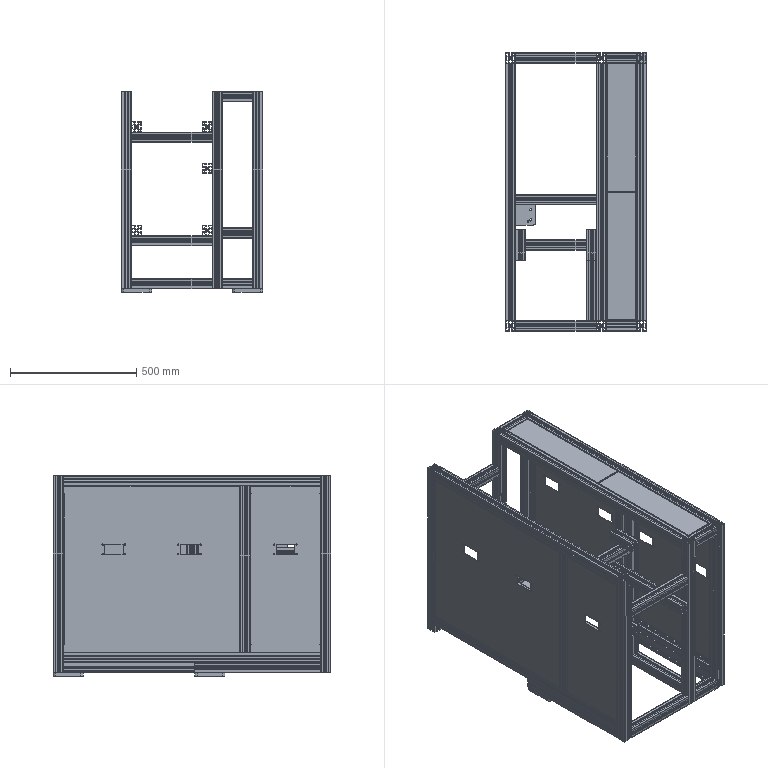Assembly | SolidWorks | mm | 41 component files | 41 solids | 3572 faces | box 560 x 1100 x 795 mm | volume 13071138 mm3 | plane 3042 | cylinder 514 | spline 16 | commonest cylinder face diameters 10.5 x170 6.8 x80 5 x56 8.5 x40 2 x36 0.762 x20 15 x20 9 x20
Bill of materials:
AluminumProfile120 | 9 | 6061 Alloy | Short straight prismatic bar with a constant square cross-section: four hollow square corner cells, a central round bore, diagonal webs, and a lengthwise slot open at the center of each of the four faces. The shortest of the profile bars in this set.
AluminumProfile320 | 6 | 6061 Alloy | Straight bar with the same four-slot square cross-section (hollow corner cells, central round bore, diagonal webs). Medium length.
AluminumProfile360 | 1 | 6061 Alloy | Straight bar with the shared four-slot square cross-section, shown with its long axis in a different orientation. Fairly long.
AluminumProfile480 | 1 | 6061 Alloy | Long straight bar with the shared four-slot square cross-section.
AluminumProfile500 | 1 | 6061 Alloy | Long straight bar with the shared four-slot square cross-section, shown in a different orientation from unnamed part.
AluminumProfile660 | 3 | 6061 Alloy | Long straight bar with the shared four-slot square cross-section, shown standing upright in the isometric view.
AluminumProfile720 | 5 | 6061 Alloy | The longest, most slender bar in the set, with the shared four-slot square cross-section.
AluminumProfile780 | 6 | 6061 Alloy | Long upright bar with the shared four-slot square cross-section, a little more slender than unnamed part.
AluminumProfileHFS8-4080Length720 | 1 | 1060 Alloy | Long straight prismatic bar with a constant rectangular cross-section, about 1:2 in aspect. The profile is a slotted extrusion-style section: two undercut T-shaped slots on each long side, one on each short side, two round center bores, an enclosed central cavity and four corner cavities.
CasterFixingPlate3 | 2 |  | Flat, thick square plate with rounded corners and nine plain round through-holes in two sizes, arranged in an asymmetric pattern.
SheetMetal120x510 | 2 |  | Long, shallow, thin-walled rectangular tray or cover: a flat, featureless top panel with short downturned flanges on all four edges. The flanges have open slots with rounded ends cut up from their free edges.
ThreeLowRackSidePlate1 | 2 | AISI 304 | Thin, flat rectangular panel, taller than it is wide (about 0.74:1). It has two rectangular through-cutouts side by side in the upper half, each with four small holes at its corners. Narrow edge returns or flanges run along two opposite edges.
ThreeLowRackSidePlate2 | 1 | AISI 304 | Thin, flat rectangular panel, a little wider than it is tall (about 1.06:1). Its features match unnamed part: two rectangular cutouts with four corner holes each, and narrow edge returns on two opposite edges.
ThreeLowRackSidePlate3 | 1 | AISI 304 | Thin, tall rectangular sheet-style panel with short bent-over flanges along its edges. It has one rectangular through-cutout centered side to side in the upper-middle area, with four small holes, one near each corner of the cutout.
Mates:
1. coincident | assembly face at (-24.557, -21.948, 2030) dir (-1, 0, 0) | assembly face at (-24.557, -1661.948, 1170) dir (-1, 0, 0)
2. coincident | assembly face at (-24.557, -21.948, 2030) dir (0, -1, 0) | assembly face at (15.443, -21.948, 1170) dir (0, 1, 0)
3. coincident | assembly face at (78.108, 18.052, 1170) dir (0, 0, 1) | assembly face at (-24.557, -1661.948, 1170) dir (0, 0, 1)
4. coincident | assembly face at (-24.557, -21.948, 2030) dir (-1, 0, 0) | assembly face at (-24.557, 898.052, 590) dir (-1, 0, 0)
5. coincident | assembly face at (-24.557, -21.948, 2030) dir (0, -1, 0) | assembly face at (15.443, -21.948, 692.665) dir (0, 1, 0)
6. distance | assembly face at (-24.557, 898.052, 630) dir (0, 0, 1) | assembly face at (-24.557, -1661.948, 1130) dir (0, 0, -1)
7. coincident | assembly face at (-24.557, -1661.948, 1170) dir (-1, 0, 0) | assembly face at (-24.557, -781.948, 2090) dir (-1, 0, 0)
8. coincident | assembly face at (-24.557, -1661.948, 1170) dir (0, 0, 1) | assembly face at (78.108, -741.948, 1170) dir (0, 0, 1)
9. coincident | assembly face at (15.443, -741.948, 1067.335) dir (0, -1, 0) | assembly face at (-24.557, -741.948, 2090) dir (0, 1, 0)
10. coincident | assembly face at (-24.557, -21.948, 2030) dir (0, -1, 0) | assembly face at (-1664.557, -21.948, 1130) dir (0, -1, 0)
11. coincident | assembly face at (-24.557, -21.948, 2030) dir (-1, 0, 0) | assembly face at (-24.557, 18.052, 1170) dir (1, 0, 0)
12. coincident | assembly face at (-24.557, -1661.948, 1170) dir (0, 0, 1) | assembly face at (-1664.557, 18.052, 1170) dir (0, 0, 1)
13. coincident | assembly face at (-24.557, -781.948, 2090) dir (0, -1, 0) | assembly face at (-1664.557, -781.948, 590) dir (0, -1, 0)
14. coincident | assembly face at (-24.557, -781.948, 2090) dir (-1, 0, 0) | assembly face at (-24.557, -741.948, 590) dir (1, 0, 0)
15. coincident | assembly face at (-24.557, 898.052, 630) dir (0, 0, 1) | assembly face at (-1664.557, -781.948, 630) dir (0, 0, 1)
16. coincident | assembly face at (-24.557, -781.948, 2090) dir (-1, 0, 0) | assembly face at (-24.557, 18.052, 527.335) dir (1, 0, 0)
17. coincident | assembly face at (-24.557, -21.948, 2030) dir (0, -1, 0) | assembly face at (1495.443, -21.948, 630) dir (0, -1, 0)
18. coincident | assembly face at (-24.557, 898.052, 630) dir (0, 0, 1) | assembly face at (1495.443, -21.948, 630) dir (0, 0, 1)
19. coincident | assembly face at (-24.557, -781.948, 2090) dir (0, -1, 0) | assembly face at (1495.443, -781.948, 1170) dir (0, -1, 0)
20. coincident | assembly face at (-24.557, -781.948, 2090) dir (-1, 0, 0) | assembly face at (-24.557, -741.948, 1067.335) dir (1, 0, 0)
21. coincident | assembly face at (-24.557, -1661.948, 1170) dir (0, 0, 1) | assembly face at (1495.443, -781.948, 1170) dir (0, 0, 1)
22. coincident | assembly face at (-1664.557, 18.052, 1170) dir (0, 0, 1) | assembly face at (-81.892, 18.052, 1170) dir (0, 0, 1)
23. coincident | assembly face at (-144.557, -84.613, 1170) dir (-1, 0, 0) | assembly face at (-144.557, -21.948, 2030) dir (1, 0, 0)
24. coincident | assembly face at (-1664.557, -21.948, 1130) dir (0, -1, 0) | assembly face at (-184.557, -21.948, 2030) dir (0, -1, 0)
25. coincident | assembly face at (-144.557, -741.948, 692.665) dir (-1, 0, 0) | assembly face at (-144.557, -781.948, 2030) dir (1, 0, 0)
26. coincident | assembly face at (-1664.557, -781.948, 590) dir (0, -1, 0) | assembly face at (-184.557, -781.948, 2030) dir (0, -1, 0)
27. coincident | assembly face at (1495.443, -781.948, 1170) dir (0, 0, 1) | assembly face at (-81.892, -741.948, 1170) dir (0, 0, 1)
28. coincident | assembly face at (-184.557, -741.948, 2030) dir (0, 1, 0) | assembly face at (-144.557, -741.948, 527.335) dir (0, -1, 0)
29. coincident | assembly face at (-184.557, -781.948, 2030) dir (-1, 0, 0) | assembly face at (-184.557, -1661.948, 630) dir (-1, 0, 0)
30. coincident | assembly face at (-1664.557, -781.948, 630) dir (0, 0, 1) | assembly face at (-184.557, -1661.948, 630) dir (0, 0, 1)
31. coincident | assembly face at (-184.557, -21.948, 2030) dir (-1, 0, 0) | assembly face at (-184.557, 898.052, 1170) dir (-1, 0, 0)
32. coincident | assembly face at (-184.557, -21.948, 2030) dir (0, -1, 0) | assembly face at (-81.892, -21.948, 1130) dir (0, 1, 0)
33. coincident | assembly face at (-1664.557, 18.052, 1170) dir (0, 0, 1) | assembly face at (-184.557, 898.052, 1170) dir (0, 0, 1)
34. coincident | assembly face at (-184.557, -781.948, 2030) dir (-1, 0, 0) | assembly face at (-184.557, -741.948, 590) dir (1, 0, 0)
35. coincident | assembly face at (-184.557, -781.948, 2030) dir (0, -1, 0) | assembly face at (-1824.557, -781.948, 590) dir (0, -1, 0)
36. coincident | assembly face at (-184.557, -1661.948, 630) dir (0, 0, 1) | assembly face at (-1824.557, -781.948, 630) dir (0, 0, 1)
37. coincident | assembly face at (-184.557, -21.948, 2030) dir (-1, 0, 0) | assembly face at (-184.557, 18.052, 630) dir (1, 0, 0)
38. coincident | assembly face at (-184.557, -21.948, 2030) dir (0, -1, 0) | assembly face at (-1824.557, -21.948, 590) dir (0, -1, 0)
39. coincident | assembly face at (-184.557, -1661.948, 630) dir (0, 0, 1) | assembly face at (-1824.557, 18.052, 630) dir (0, 0, 1)
40. coincident | assembly face at (-184.557, -21.948, 2030) dir (-1, 0, 0) | assembly face at (-184.557, 18.052, 970) dir (1, 0, 0)
41. coincident | assembly face at (-184.557, -21.948, 2030) dir (0, -1, 0) | assembly face at (-1824.557, -21.948, 970) dir (0, -1, 0)
42. distance | assembly face at (-1664.557, 18.052, 1170) dir (0, 0, 1) | assembly face at (-1824.557, -21.948, 1010) dir (0, 0, 1)
43. coincident | assembly face at (-184.557, -781.948, 2030) dir (0, -1, 0) | assembly face at (-1824.557, -781.948, 970) dir (0, -1, 0)
44. coincident | assembly face at (-184.557, -781.948, 2030) dir (-1, 0, 0) | assembly face at (-184.557, -741.948, 1010) dir (1, 0, 0)
45. distance | assembly face at (-184.557, 898.052, 1170) dir (0, 0, 1) | assembly face at (-1824.557, -741.948, 1010) dir (0, 0, 1)
46. coincident | assembly face at (-184.557, -21.948, 2030) dir (-1, 0, 0) | assembly face at (-184.557, 1578.052, 1050) dir (1, 0, 0)
47. coincident | assembly face at (-1824.557, -21.948, 1010) dir (0, 0, 1) | assembly face at (-224.557, 1578.052, 1010) dir (0, 0, -1)
48. distance | assembly face at (-224.557, -61.948, 1010) dir (0, -1, 0) | assembly face at (-1824.557, -21.948, 970) dir (0, -1, 0)
49. coincident | assembly face at (-464.557, 18.052, 1072.665) dir (-1, 0, 0) | assembly face at (-464.557, -1581.948, 1010) dir (-1, 0, 0)
50. coincident | assembly face at (-1824.557, -21.948, 1010) dir (0, 0, 1) | assembly face at (-464.557, -1581.948, 1010) dir (0, 0, -1)
51. distance | assembly face at (-464.557, 58.052, 1050) dir (0, 1, 0) | assembly face at (-1824.557, 18.052, 970) dir (0, 1, 0)
52. coincident | assembly face at (-184.557, -781.948, 2030) dir (-1, 0, 0) | assembly face at (-184.557, -2341.948, 1010) dir (1, 0, 0)
53. coincident | assembly face at (-1824.557, -741.948, 1010) dir (0, 0, 1) | assembly face at (-224.557, -2341.948, 1010) dir (0, 0, -1)
54. distance | assembly face at (-224.557, -701.948, 1050) dir (0, 1, 0) | assembly face at (-1824.557, -741.948, 970) dir (0, 1, 0)
55. coincident | assembly face at (-464.557, -844.613, 1010) dir (-1, 0, 0) | assembly face at (-464.557, 818.052, 1010) dir (-1, 0, 0)
56. coincident | assembly face at (-1824.557, -741.948, 1010) dir (0, 0, 1) | assembly face at (-464.557, 818.052, 1010) dir (0, 0, -1)
57. distance | assembly face at (-424.557, -821.948, 1010) dir (0, -1, 0) | assembly face at (-1824.557, -781.948, 970) dir (0, -1, 0)
58. coincident | assembly face at (-184.557, -21.948, 2030) dir (-1, 0, 0) | assembly face at (-184.557, -1581.948, 630) dir (1, 0, 0)
59. coincident | assembly face at (-1824.557, 18.052, 630) dir (0, 0, 1) | assembly face at (-184.557, -1581.948, 630) dir (0, 0, -1)
60. distance | assembly face at (-1824.557, 18.052, 590) dir (0, 1, 0) | assembly face at (-224.557, 58.052, 630) dir (0, 1, 0)
61. coincident | assembly face at (-464.557, -84.613, 630) dir (-1, 0, 0) | assembly face at (-464.557, -1581.948, 630) dir (-1, 0, 0)
62. coincident | assembly face at (-1824.557, 18.052, 630) dir (0, 0, 1) | assembly face at (-464.557, -1581.948, 630) dir (0, 0, -1)
63. distance | assembly face at (-464.557, 58.052, 670) dir (0, 1, 0) | assembly face at (-1824.557, 18.052, 590) dir (0, 1, 0)
64. coincident | assembly face at (-184.557, -781.948, 2030) dir (-1, 0, 0) | assembly face at (-184.557, 818.052, 630) dir (1, 0, 0)
65. coincident | assembly face at (-1824.557, -781.948, 630) dir (0, 0, 1) | assembly face at (-224.557, 818.052, 630) dir (0, 0, -1)
66. distance | assembly face at (-1824.557, -781.948, 590) dir (0, -1, 0) | assembly face at (-184.557, -821.948, 630) dir (0, -1, 0)
67. coincident | assembly face at (-464.557, -741.948, 692.665) dir (-1, 0, 0) | assembly face at (-464.557, -2341.948, 630) dir (-1, 0, 0)
68. coincident | assembly face at (-1824.557, -781.948, 630) dir (0, 0, 1) | assembly face at (-464.557, -2341.948, 630) dir (0, 0, -1)
69. distance | assembly face at (-1824.557, -741.948, 590) dir (0, 1, 0) | assembly face at (-464.557, -701.948, 670) dir (0, 1, 0)
70. coincident | assembly face at (-464.557, -1581.948, 1010) dir (-1, 0, 0) | assembly face at (-464.557, -21.948, 2390) dir (-1, 0, 0)
71. coincident | assembly face at (-1824.557, -21.948, 970) dir (0, -1, 0) | assembly face at (-464.557, -21.948, 2390) dir (0, -1, 0)
72. coincident | assembly face at (-1824.557, -21.948, 970) dir (0, 0, -1) | assembly face at (-361.892, 18.052, 970) dir (0, 0, 1)
73. coincident | assembly face at (-464.557, -844.613, 1010) dir (-1, 0, 0) | assembly face at (-464.557, -781.948, 2390) dir (-1, 0, 0)
74. coincident | assembly face at (-1824.557, -781.948, 970) dir (0, -1, 0) | assembly face at (-464.557, -781.948, 2390) dir (0, -1, 0)
75. coincident | assembly face at (-1824.557, -741.948, 970) dir (0, 0, -1) | assembly face at (-361.892, -741.948, 970) dir (0, 0, 1)
76. coincident | assembly face at (-464.557, -741.948, 692.665) dir (-1, 0, 0) | assembly face at (-464.557, -781.948, 2030) dir (-1, 0, 0)
77. coincident | assembly face at (-1824.557, -781.948, 590) dir (0, -1, 0) | assembly face at (-464.557, -781.948, 2030) dir (0, -1, 0)
78. coincident | assembly face at (-1824.557, -781.948, 590) dir (0, 0, -1) | assembly face at (-361.892, -741.948, 590) dir (0, 0, 1)
79. coincident | assembly face at (-464.557, -84.613, 630) dir (-1, 0, 0) | assembly face at (-464.557, -21.948, 2030) dir (-1, 0, 0)
80. coincident | assembly face at (-1824.557, 18.052, 590) dir (0, 1, 0) | assembly face at (-464.557, 18.052, 2030) dir (0, 1, 0)
81. coincident | assembly face at (-1824.557, 18.052, 590) dir (0, 0, -1) | assembly face at (-361.892, 18.052, 590) dir (0, 0, 1)
82. coincident | assembly face at (-24.557, -741.948, 1067.335) dir (1, 0, 0) | assembly face at (-24.557, -781.948, 2030) dir (-1, 0, 0)
83. coincident | assembly face at (1495.443, -781.948, 1170) dir (0, -1, 0) | assembly face at (-24.557, -781.948, 2030) dir (0, -1, 0)
84. coincident | assembly face at (1495.443, -781.948, 1170) dir (0, 0, 1) | assembly face at (78.108, -741.948, 1170) dir (0, 0, 1)
85. coincident | assembly face at (15.443, -781.948, 2030) dir (1, 0, 0) | assembly face at (15.443, -631.948, 375) dir (1, 0, 0)
86. coincident | assembly face at (-24.557, -781.948, 2030) dir (0, -1, 0) | assembly face at (15.443, -781.948, 375) dir (0, -1, 0)
87. coincident | assembly face at (-24.557, -741.948, 390) dir (0, 0, -1) | assembly face at (15.443, -631.948, 390) dir (0, 0, 1)
88. coincident | assembly face at (15.443, -21.948, 2030) dir (1, 0, 0) | assembly face at (15.443, 18.052, 375) dir (1, 0, 0)
89. coincident | assembly face at (-24.557, 18.052, 2030) dir (0, 1, 0) | assembly face at (15.443, 18.052, 375) dir (0, 1, 0)
90. coincident | assembly face at (-24.557, 18.052, 390) dir (0, 0, -1) | assembly face at (15.443, 18.052, 390) dir (0, 0, 1)
91. coincident | assembly face at (-464.557, -21.948, 2030) dir (-1, 0, 0) | assembly face at (-464.557, -131.948, 375) dir (-1, 0, 0)
92. coincident | assembly face at (-464.557, 18.052, 2030) dir (0, 1, 0) | assembly face at (-464.557, 18.052, 375) dir (0, 1, 0)
93. coincident | assembly face at (-464.557, 18.052, 390) dir (0, 0, -1) | assembly face at (-464.557, -131.948, 390) dir (0, 0, 1)
94. coincident | assembly face at (-464.557, -781.948, 2030) dir (0, -1, 0) | assembly face at (-464.557, -781.948, 375) dir (0, -1, 0)
95. coincident | assembly face at (-464.557, -781.948, 2030) dir (-1, 0, 0) | assembly face at (-464.557, -781.948, 375) dir (-1, 0, 0)
96. coincident | assembly face at (-464.557, -741.948, 390) dir (0, 0, -1) | assembly face at (-464.557, -781.948, 390) dir (0, 0, 1)
97. coincident | assembly face at (-24.557, -741.948, 590) dir (1, 0, 0) | assembly face at (-24.557, -781.948, 2030) dir (-1, 0, 0)
98. coincident | assembly face at (-184.557, -781.948, 2030) dir (-1, 0, 0) | assembly face at (-184.557, 898.052, 1170) dir (-1, 0, 0)
99. coincident | assembly face at (1495.443, -781.948, 1170) dir (0, -1, 0) | assembly face at (-184.557, -781.948, 2030) dir (0, -1, 0)
100. coincident | assembly face at (15.443, -741.948, 1067.335) dir (0, -1, 0) | assembly face at (-24.557, -741.948, 2030) dir (0, 1, 0)
101. coincident | assembly face at (-184.557, -1661.948, 630) dir (-1, 0, 0) | assembly face at (-184.557, 898.052, 1170) dir (-1, 0, 0)
102. coincident | assembly face at (1495.443, -21.948, 630) dir (0, 0, 1) | assembly face at (-184.557, -1661.948, 630) dir (0, 0, 1)
103. distance | assembly face at (-184.557, -1661.948, 590) dir (0, 0, -1) | assembly face at (-24.557, -741.948, 390) dir (0, 0, -1)
104. coincident | assembly face at (-24.557, -741.948, 2030) dir (0, 1, 0) | assembly face at (-4.557, -741.948, 430) dir (0, -1, 0)
105. coincident | assembly face at (15.443, -781.948, 2030) dir (1, 0, 0) | assembly face at (15.443, -741.948, 415.3) dir (1, 0, 0)
106. coincident | assembly face at (-24.557, -741.948, 390) dir (0, 0, -1) | assembly face at (0.7428, -741.948, 390) dir (0, 0, -1)
107. coincident | AluminumProfile780-1 face at (-768.352, 51.783, 1543.715) dir (-1, 0, 0) | AluminumProfile720-1 face at (-768.352, 671.783, 643.715) dir (-1, 0, 0)
108. coincident | AluminumProfile780-1 face at (-768.352, 51.783, 1543.715) dir (0, -1, 0) | AluminumProfile720-1 face at (-831.017, 51.783, 683.715) dir (0, 1, 0)
109. coincident | AluminumProfile780-1 face at (-665.687, 91.783, 683.715) dir (0, 0, 1) | AluminumProfile720-1 face at (-728.352, 671.783, 683.715) dir (0, 0, 1)
110. coincident | AluminumProfile780-1 face at (-768.352, 51.783, 1543.715) dir (0, -1, 0) | assembly face at (-748.352, 51.783, -56.285) dir (0, 1, 0)
111. coincident | AluminumProfile780-1 face at (-768.352, 51.783, 1543.715) dir (-1, 0, 0) | assembly face at (-768.352, 51.783, -70.985) dir (-1, 0, 0)
112. coincident | AluminumProfile780-1 face at (-768.352, 91.783, -96.285) dir (0, 0, -1) | assembly face at (-753.652, 51.783, -96.285) dir (0, 0, -1)
113. coincident | AluminumProfile720-1 face at (-728.352, -968.217, 683.715) dir (0, -1, 0) | AluminumProfile780-2 face at (-768.352, -968.217, 1543.715) dir (0, 1, 0)
114. coincident | AluminumProfile720-1 face at (-768.352, 671.783, 643.715) dir (-1, 0, 0) | AluminumProfile780-2 face at (-768.352, -1008.217, 1543.715) dir (-1, 0, 0)
115. coincident | AluminumProfile720-1 face at (-728.352, 671.783, 683.715) dir (0, 0, 1) | AluminumProfile780-2 face at (-665.687, -968.217, 683.715) dir (0, 0, 1)
116. coincident | AluminumProfile780-1 face at (-768.352, 51.783, 1543.715) dir (0, -1, 0) | AluminumProfileHFS8-4080Length720-2 face at (-748.352, 51.783, -56.285) dir (0, 1, 0)
117. coincident | AluminumProfile780-1 face at (-768.352, 51.783, 1543.715) dir (-1, 0, 0) | AluminumProfileHFS8-4080Length720-2 face at (-768.352, 51.783, -70.985) dir (-1, 0, 0)
118. coincident | AluminumProfile780-1 face at (-768.352, 91.783, -96.285) dir (0, 0, -1) | AluminumProfileHFS8-4080Length720-2 face at (-753.652, 51.783, -96.285) dir (0, 0, -1)
119. coincident | AluminumProfile780-1 face at (-768.352, 51.783, 1543.715) dir (-1, 0, 0) | AluminumProfile120-1 face at (-768.352, 91.783, 643.715) dir (1, 0, 0)
120. coincident | AluminumProfile720-1 face at (-728.352, 671.783, 683.715) dir (0, 0, 1) | AluminumProfile120-1 face at (-2408.352, 51.783, 683.715) dir (0, 0, 1)
121. coincident | AluminumProfile780-1 face at (-768.352, 91.783, 1543.715) dir (0, 1, 0) | AluminumProfile120-1 face at (-2408.352, 91.783, 643.715) dir (0, 1, 0)
122. coincident | AluminumProfileHFS8-4080Length720-2 face at (-768.352, 51.783, -70.985) dir (-1, 0, 0) | AluminumProfile120-2 face at (-768.352, -1008.217, 643.715) dir (1, 0, 0)
123. coincident | AluminumProfile720-1 face at (-728.352, 671.783, 683.715) dir (0, 0, 1) | AluminumProfile120-2 face at (-2408.352, -1008.217, 683.715) dir (0, 0, 1)
124. coincident | AluminumProfile780-2 face at (-768.352, -1008.217, 1543.715) dir (0, -1, 0) | AluminumProfile120-2 face at (-2408.352, -1008.217, 683.715) dir (0, -1, 0)
125. coincident | AluminumProfile780-1 face at (-768.352, 51.783, 1543.715) dir (-1, 0, 0) | AluminumProfile120-3 face at (-768.352, 91.783, 143.715) dir (1, 0, 0)
126. coincident | AluminumProfile780-1 face at (-768.352, 51.783, 1543.715) dir (0, -1, 0) | AluminumProfile120-3 face at (-2408.352, 51.783, 103.715) dir (0, -1, 0)
127. distance | AluminumProfileHFS8-4080Length720-2 face at (-753.652, 51.783, -96.285) dir (0, 0, -1) | AluminumProfile120-3 face at (-2408.352, 91.783, 103.715) dir (0, 0, -1)
128. coincident | AluminumProfile780-2 face at (-768.352, -1008.217, 1543.715) dir (-1, 0, 0) | AluminumProfile120-4 face at (-768.352, -968.217, -158.95) dir (1, 0, 0)
129. coincident | AluminumProfile780-2 face at (-768.352, -1008.217, 1543.715) dir (0, -1, 0) | AluminumProfile120-4 face at (751.648, -1008.217, -56.285) dir (0, -1, 0)
130. coincident | AluminumProfileHFS8-4080Length720-2 face at (-753.652, 51.783, -96.285) dir (0, 0, -1) | AluminumProfile120-4 face at (751.648, -1008.217, -96.285) dir (0, 0, -1)
131. coincident | AluminumProfile120-4 face at (751.648, -1008.217, -56.285) dir (0, -1, 0) | AluminumProfile780-3 face at (-928.352, -1008.217, 1543.715) dir (0, -1, 0)
132. coincident | AluminumProfile120-4 face at (-888.352, -968.217, -56.285) dir (-1, 0, 0) | AluminumProfile780-3 face at (-888.352, -1008.217, 1543.715) dir (1, 0, 0)
133. coincident | AluminumProfile120-2 face at (-2408.352, -1008.217, 683.715) dir (0, 0, 1) | AluminumProfile780-3 face at (-825.687, -968.217, 683.715) dir (0, 0, 1)
134. coincident | AluminumProfile120-3 face at (-888.352, -10.882, 143.715) dir (-1, 0, 0) | AluminumProfile780-4 face at (-888.352, 51.783, 1543.715) dir (1, 0, 0)
135. coincident | AluminumProfile120-3 face at (-2408.352, 91.783, 103.715) dir (0, 1, 0) | AluminumProfile780-4 face at (-928.352, 91.783, 1543.715) dir (0, 1, 0)
136. coincident | AluminumProfile120-1 face at (-2408.352, 51.783, 683.715) dir (0, 0, 1) | AluminumProfile780-4 face at (-825.687, 91.783, 683.715) dir (0, 0, 1)
137. coincident | AluminumProfile780-3 face at (-928.352, -968.217, 1543.715) dir (0, 1, 0) | AluminumProfile720-2 face at (-825.687, -968.217, 683.715) dir (0, -1, 0)
138. coincident | AluminumProfile780-3 face at (-928.352, -1008.217, 1543.715) dir (-1, 0, 0) | AluminumProfile720-2 face at (-928.352, -1588.217, 643.715) dir (-1, 0, 0)
139. coincident | AluminumProfile120-2 face at (-2408.352, -1008.217, 683.715) dir (0, 0, 1) | AluminumProfile720-2 face at (-928.352, -1588.217, 683.715) dir (0, 0, 1)
140. coincident | AluminumProfile780-4 face at (-928.352, 51.783, 1543.715) dir (0, -1, 0) | assembly face at (-928.352, 51.783, 143.715) dir (0, 1, 0)
141. coincident | AluminumProfile780-3 face at (-928.352, -1008.217, 1543.715) dir (-1, 0, 0) | assembly face at (-928.352, -1588.217, 103.715) dir (-1, 0, 0)
142. coincident | AluminumProfile120-4 face at (751.648, -1008.217, -96.285) dir (0, 0, -1) | assembly face at (-928.352, -1588.217, 103.715) dir (0, 0, -1)
143. coincident | AluminumProfile780-3 face at (-928.352, -1008.217, 1543.715) dir (0, -1, 0) | assembly face at (311.648, -708.217, 143.715) dir (0, -1, 0)
144. coincident | AluminumProfile780-3 face at (-928.352, -1008.217, 1543.715) dir (-1, 0, 0) | assembly face at (-928.352, -668.217, 41.05) dir (1, 0, 0)
145. coincident | AluminumProfile120-4 face at (751.648, -1008.217, -56.285) dir (0, 0, 1) | assembly face at (311.648, -708.217, 143.715) dir (0, 0, 1)
146. coincident | AluminumProfile780-3 face at (-928.352, -1008.217, 1543.715) dir (-1, 0, 0) | assembly face at (-928.352, 946.601, 143.715) dir (1, 0, 0)
147. distance | assembly face at (-928.352, -748.217, 143.715) dir (0, -1, 0) | assembly face at (311.648, -708.217, 143.715) dir (0, -1, 0)
148. coincident | assembly face at (311.648, -708.217, 143.715) dir (0, 0, 1) | assembly face at (-968.352, 891.783, 143.715) dir (0, 0, -1)
149. coincident | assembly face at (-928.352, -693.399, 143.715) dir (0, -1, 0) | assembly face at (-1105.687, -693.399, 183.715) dir (0, -1, 0)
150. coincident | assembly face at (-968.352, 946.601, 183.715) dir (0, 0, 1) | assembly face at (-1208.352, -2213.399, 183.715) dir (0, 0, 1)
151. distance | assembly face at (-968.352, 946.601, 143.715) dir (-1, 0, 0) | assembly face at (-1168.352, -2213.399, 143.715) dir (1, 0, 0)
152. coincident | AluminumProfile780-3 face at (-928.352, -1008.217, 1543.715) dir (-1, 0, 0) | assembly face at (-928.352, -668.217, 523.715) dir (1, 0, 0)
153. coincident | AluminumProfile780-3 face at (-928.352, -1008.217, 1543.715) dir (0, -1, 0) | assembly face at (-2568.352, -708.217, 483.715) dir (0, -1, 0)
154. distance | AluminumProfile720-2 face at (-928.352, -1588.217, 683.715) dir (0, 0, 1) | assembly face at (-2568.352, -668.217, 523.715) dir (0, 0, 1)
155. coincident | assembly face at (-928.352, -748.217, 143.715) dir (0, -1, 0) | assembly face at (-865.687, -748.217, 563.715) dir (0, -1, 0)
156. coincident | AluminumProfile780-3 face at (-928.352, -1008.217, 1543.715) dir (-1, 0, 0) | assembly face at (-928.352, -2268.217, 523.715) dir (1, 0, 0)
157. coincident | assembly face at (-2568.352, -668.217, 523.715) dir (0, 0, 1) | assembly face at (-968.352, -2268.217, 523.715) dir (0, 0, -1)
158. coincident | assembly face at (-865.687, -748.217, 563.715) dir (0, -1, 0) | assembly face at (-1208.352, -748.217, 626.38) dir (0, -1, 0)
159. coincident | assembly face at (-968.352, -2268.217, 563.715) dir (0, 0, 1) | assembly face at (-1168.352, -2268.217, 563.715) dir (0, 0, 1)
160. distance | assembly face at (-968.352, -2268.217, 523.715) dir (-1, 0, 0) | assembly face at (-1168.352, -2268.217, 523.715) dir (1, 0, 0)
161. coincident | AluminumProfile780-3 face at (-928.352, -1008.217, 1543.715) dir (0, -1, 0) | AluminumProfile320-1 face at (-2568.352, -1008.217, -96.285) dir (0, -1, 0)
162. coincident | AluminumProfile780-3 face at (-928.352, -1008.217, 1543.715) dir (-1, 0, 0) | AluminumProfile320-1 face at (-928.352, -968.217, -56.285) dir (1, 0, 0)
163. coincident | AluminumProfile780-3 face at (-928.352, -1008.217, 1543.715) dir (0, -1, 0) | AluminumProfile320-2 face at (-2568.352, -1008.217, 483.715) dir (0, -1, 0)
164. coincident | AluminumProfile780-3 face at (-928.352, -1008.217, 1543.715) dir (-1, 0, 0) | AluminumProfile320-2 face at (-928.352, -968.217, 523.715) dir (1, 0, 0)
165. distance | AluminumProfile720-2 face at (-928.352, -1588.217, 683.715) dir (0, 0, 1) | AluminumProfile320-2 face at (-2568.352, -968.217, 523.715) dir (0, 0, 1)
166. coincident | AluminumProfile780-4 face at (-928.352, 91.783, 1543.715) dir (0, 1, 0) | AluminumProfile320-3 face at (-2568.352, 91.783, -96.285) dir (0, 1, 0)
167. coincident | AluminumProfile780-4 face at (-928.352, 51.783, 1543.715) dir (-1, 0, 0) | AluminumProfile320-3 face at (-928.352, 91.783, -96.285) dir (1, 0, 0)
168. coincident | AluminumProfile780-4 face at (-928.352, 51.783, 1543.715) dir (-1, 0, 0) | AluminumProfile320-4 face at (-928.352, 91.783, 483.715) dir (1, 0, 0)
169. coincident | AluminumProfile780-4 face at (-928.352, 91.783, 1543.715) dir (0, 1, 0) | AluminumProfile320-4 face at (-2568.352, 91.783, 483.715) dir (0, 1, 0)
170. distance | AluminumProfile720-2 face at (-928.352, -1588.217, 683.715) dir (0, 0, 1) | AluminumProfile320-4 face at (-2568.352, 51.783, 523.715) dir (0, 0, 1)
171. coincident | AluminumProfile780-4 face at (-928.352, 51.783, 1543.715) dir (-1, 0, 0) | assembly face at (-928.352, -1508.217, 523.715) dir (1, 0, 0)
172. coincident | AluminumProfile320-4 face at (-2568.352, 51.783, 523.715) dir (0, 0, 1) | assembly face at (-928.352, -1508.217, 523.715) dir (0, 0, -1)
173. distance | assembly face at (-968.352, 131.783, 523.715) dir (0, 1, 0) | AluminumProfile320-4 face at (-2568.352, 91.783, 483.715) dir (0, 1, 0)
174. coincident | AluminumProfile780-3 face at (-928.352, -1008.217, 1543.715) dir (-1, 0, 0) | assembly face at (-928.352, -2268.217, 523.715) dir (1, 0, 0)
175. distance | assembly face at (-968.352, -628.217, 523.715) dir (0, 1, 0) | AluminumProfile320-2 face at (-2568.352, -968.217, 483.715) dir (0, 1, 0)
176. coincident | AluminumProfile320-2 face at (-2568.352, -968.217, 523.715) dir (0, 0, 1) | assembly face at (-928.352, -2268.217, 523.715) dir (0, 0, -1)
177. coincident | assembly face at (-968.352, -748.217, 626.38) dir (0, -1, 0) | assembly face at (-1208.352, -748.217, 626.38) dir (0, -1, 0)
178. coincident | AluminumProfile320-2 face at (-2568.352, -968.217, 523.715) dir (0, 0, 1) | assembly face at (-1168.352, -2268.217, 523.715) dir (0, 0, -1)
179. distance | assembly face at (-968.352, -2268.217, 523.715) dir (-1, 0, 0) | assembly face at (-1168.352, -2268.217, 523.715) dir (1, 0, 0)
180. coincident | AluminumProfile780-3 face at (-928.352, -1008.217, 1543.715) dir (-1, 0, 0) | assembly face at (-928.352, -2268.217, 143.715) dir (1, 0, 0)
181. coincident | AluminumProfile320-1 face at (-2568.352, -968.217, -56.285) dir (0, 0, 1) | assembly face at (-968.352, -2268.217, 143.715) dir (0, 0, -1)
182. distance | AluminumProfile320-1 face at (-2568.352, -968.217, -96.285) dir (0, 1, 0) | assembly face at (-968.352, -628.217, 183.715) dir (0, 1, 0)
183. coincident | AluminumProfile780-4 face at (-928.352, 51.783, 1543.715) dir (-1, 0, 0) | assembly face at (-928.352, -1508.217, 143.715) dir (1, 0, 0)
184. distance | assembly face at (-968.352, 131.783, 183.715) dir (0, 1, 0) | AluminumProfile320-3 face at (-2568.352, 91.783, -96.285) dir (0, 1, 0)
185. coincident | AluminumProfile320-3 face at (-2568.352, 51.783, -56.285) dir (0, 0, 1) | assembly face at (-1208.352, 1651.783, 143.715) dir (0, 0, -1)
186. distance | assembly face at (-968.352, -1508.217, 143.715) dir (-1, 0, 0) | assembly face at (-1168.352, 1651.783, 143.715) dir (1, 0, 0)
187. distance | assembly face at (-1168.352, 11.783, 143.715) dir (0, -1, 0) | AluminumProfile320-3 face at (-2568.352, 51.783, -96.285) dir (0, -1, 0)
188. coincident | AluminumProfile320-4 face at (-2568.352, 51.783, 523.715) dir (0, 0, 1) | assembly face at (-1208.352, -1508.217, 523.715) dir (0, 0, -1)
189. distance | assembly face at (-1208.352, 131.783, 563.715) dir (0, 1, 0) | AluminumProfile320-4 face at (-2568.352, 91.783, 483.715) dir (0, 1, 0)
190. distance | assembly face at (-968.352, -1508.217, 523.715) dir (-1, 0, 0) | assembly face at (-1168.352, -1508.217, 523.715) dir (1, 0, 0)
191. coincident | AluminumProfile320-1 face at (-2568.352, -968.217, -56.285) dir (0, 0, 1) | assembly face at (-1208.352, -2268.217, 143.715) dir (0, 0, -1)
192. distance | AluminumProfile320-1 face at (-2568.352, -968.217, -96.285) dir (0, 1, 0) | assembly face at (-1208.352, -628.217, 183.715) dir (0, 1, 0)
193. distance | assembly face at (-968.352, -2268.217, 143.715) dir (-1, 0, 0) | assembly face at (-1168.352, -2268.217, 143.715) dir (1, 0, 0)
194. coincident | AluminumProfile320-1 face at (-2568.352, -1008.217, -96.285) dir (0, -1, 0) | AluminumProfile780-5 face at (-1288.352, -1008.217, 1543.715) dir (0, -1, 0)
195. coincident | AluminumProfile320-1 face at (-1248.352, -1070.882, -56.285) dir (-1, 0, 0) | AluminumProfile780-5 face at (-1248.352, -1008.217, 1543.715) dir (1, 0, 0)
196. coincident | AluminumProfile780-3 face at (-928.352, -968.217, -96.285) dir (0, 0, -1) | AluminumProfile780-5 face at (-1288.352, -968.217, -96.285) dir (0, 0, -1)
197. coincident | AluminumProfile320-3 face at (-1248.352, 91.783, 6.38) dir (-1, 0, 0) | AluminumProfile780-6 face at (-1248.352, 51.783, 1543.715) dir (1, 0, 0)
198. coincident | AluminumProfile320-3 face at (-2568.352, 91.783, -96.285) dir (0, 1, 0) | AluminumProfile780-6 face at (-1288.352, 91.783, 1543.715) dir (0, 1, 0)
199. coincident | AluminumProfile780-4 face at (-928.352, 91.783, -96.285) dir (0, 0, -1) | AluminumProfile780-6 face at (-1288.352, 91.783, -96.285) dir (0, 0, -1)
200. coincident | AluminumProfile780-6 face at (-1288.352, 51.783, 1543.715) dir (0, -1, 0) | AluminumProfile720-4 face at (-1248.352, 51.783, 746.38) dir (0, 1, 0)
201. coincident | AluminumProfile780-6 face at (-1288.352, 51.783, 1543.715) dir (-1, 0, 0) | AluminumProfile720-4 face at (-1288.352, 671.783, 643.715) dir (-1, 0, 0)
202. coincident | AluminumProfile780-6 face at (-1185.687, 91.783, 683.715) dir (0, 0, 1) | AluminumProfile720-4 face at (-1288.352, 671.783, 683.715) dir (0, 0, 1)
203. coincident | AluminumProfile780-6 face at (-1288.352, 51.783, 1543.715) dir (-1, 0, 0) | assembly face at (-1288.352, 971.783, 103.715) dir (-1, 0, 0)
204. coincident | AluminumProfile780-6 face at (-1288.352, 51.783, 1543.715) dir (0, -1, 0) | assembly face at (-1248.352, 51.783, 206.38) dir (0, 1, 0)
205. coincident | AluminumProfile320-3 face at (-2568.352, 51.783, -56.285) dir (0, 0, 1) | assembly face at (-1288.352, 971.783, 143.715) dir (0, 0, 1)
206. coincident | AluminumProfile720-4 face at (-1288.352, 671.783, 643.715) dir (0, 0, -1) | assembly face at (-1185.687, -468.217, 643.715) dir (0, 0, 1)
207. coincident | AluminumProfile720-4 face at (-1288.352, 671.783, 643.715) dir (-1, 0, 0) | assembly face at (-1288.352, -508.217, 1783.715) dir (-1, 0, 0)
208. distance | AluminumProfile720-2 face at (-928.352, -1588.217, 683.715) dir (0, 0, 1) | assembly face at (-2568.352, -768.217, 523.715) dir (0, 0, 1)
209. coincident | assembly face at (-2568.352, -768.217, 523.715) dir (0, 0, 1) | assembly face at (-968.352, 791.783, 523.715) dir (0, 0, -1)
210. distance | assembly face at (-2568.352, -808.217, 483.715) dir (0, -1, 0) | assembly face at (-928.352, -848.217, 523.715) dir (0, -1, 0)
211. coincident | assembly face at (-928.352, -1588.217, 103.715) dir (-1, 0, 0) | assembly face at (-928.352, -2368.217, 143.715) dir (1, 0, 0)
212. coincident | assembly face at (-2568.352, -768.217, 143.715) dir (0, 0, 1) | assembly face at (-928.352, -2368.217, 143.715) dir (0, 0, -1)
213. distance | assembly face at (-968.352, -728.217, 143.715) dir (0, 1, 0) | assembly face at (-2568.352, -768.217, 103.715) dir (0, 1, 0)
214. distance | assembly face at (-968.352, -2368.217, 143.715) dir (-1, 0, 0) | assembly face at (-1168.352, -2368.217, 143.715) dir (1, 0, 0)
215. coincident | assembly face at (-968.352, 791.783, 563.715) dir (0, 0, 1) | assembly face at (-1208.352, -2368.217, 563.715) dir (0, 0, 1)
216. coincident | assembly face at (-928.352, -848.217, 523.715) dir (0, -1, 0) | assembly face at (-1105.687, -848.217, 563.715) dir (0, -1, 0)
217. coincident | assembly face at (-1168.352, -2147.847, 143.715) dir (1, 0, 0) | assembly face at (-1168.352, -2368.217, 523.715) dir (1, 0, 0)
218. coincident | assembly face at (-928.352, -1588.217, 103.715) dir (0, 0, -1) | assembly face at (-2568.352, -653.542, 103.715) dir (0, 0, -1)
219. coincident | AluminumProfile720-6 face at (-1248.352, -968.217, -56.285) dir (0, -1, 0) | AluminumProfile780-5 face at (-1288.352, -968.217, 1543.715) dir (0, 1, 0)
220. coincident | AluminumProfile780-5 face at (-1288.352, -1008.217, 1543.715) dir (-1, 0, 0) | AluminumProfile720-6 face at (-1288.352, 671.783, -56.285) dir (-1, 0, 0)
221. distance | AluminumProfile780-6 face at (-1288.352, 91.783, -96.285) dir (0, 0, -1) | AluminumProfile720-6 face at (-1288.352, 671.783, -56.285) dir (0, 0, -1)
222. coincident | AluminumProfile720-4 face at (-1288.352, 671.783, 643.715) dir (0, 0, -1) | AluminumProfile660-1 face at (-1185.687, -648.217, 643.715) dir (0, 0, 1)
223. coincident | AluminumProfile720-4 face at (-1288.352, 671.783, 643.715) dir (-1, 0, 0) | AluminumProfile660-1 face at (-1288.352, -688.217, 1623.715) dir (-1, 0, 0)
224. coincident | assembly face at (-2568.352, -547.847, 143.715) dir (0, 0, 1) | assembly face at (-1208.352, -2147.847, 143.715) dir (0, 0, -1)
225. coincident | assembly face at (-968.352, -627.847, 246.38) dir (0, -1, 0) | assembly face at (-1105.687, -627.847, 183.715) dir (0, -1, 0)
226. coincident | assembly face at (-928.352, -1588.217, 103.715) dir (-1, 0, 0) | assembly face at (-928.352, -653.542, 143.715) dir (1, 0, 0)
227. coincident | AluminumProfile780-4 face at (-928.352, 51.783, 1543.715) dir (0, -1, 0) | AluminumProfile720-7 face at (-888.352, 51.783, -16.285) dir (0, 1, 0)
228. coincident | AluminumProfile780-3 face at (-888.352, -1008.217, 1543.715) dir (1, 0, 0) | AluminumProfile720-7 face at (-888.352, -1588.217, -16.285) dir (1, 0, 0)
229. coincident | AluminumProfileHFS8-4080Length720-2 face at (-765.352, 51.783, -16.285) dir (0, 0, 1) | AluminumProfile720-7 face at (-928.352, -1588.217, -16.285) dir (0, 0, 1)
230. coincident | AluminumProfile720-2 face at (-928.352, -1588.217, 643.715) dir (0, 0, -1) | AluminumProfile660-2 face at (-825.687, -648.217, 643.715) dir (0, 0, 1)
231. coincident | AluminumProfile720-2 face at (-928.352, -1588.217, 643.715) dir (-1, 0, 0) | AluminumProfile660-2 face at (-928.352, -688.217, 1623.715) dir (-1, 0, 0)
232. distance | AluminumProfile660-2 face at (-928.352, -688.217, 1623.715) dir (0, -1, 0) | AluminumProfile780-3 face at (-928.352, -968.217, 1543.715) dir (0, 1, 0)
233. coincident | AluminumProfile660-1 face at (-1248.352, -688.217, 1623.715) dir (1, 0, 0) | AluminumProfile320-7 face at (-1248.352, -750.882, 113.715) dir (-1, 0, 0)
234. coincident | AluminumProfile660-1 face at (-1288.352, -688.217, 1623.715) dir (0, -1, 0) | AluminumProfile320-7 face at (-2568.352, -688.217, 73.715) dir (0, -1, 0)
235. coincident | AluminumProfile660-1 face at (-1248.352, -688.217, 1623.715) dir (1, 0, 0) | AluminumProfile320-8 face at (-1248.352, -688.217, 523.715) dir (-1, 0, 0)
236. coincident | AluminumProfile660-1 face at (-1288.352, -688.217, 1623.715) dir (0, -1, 0) | AluminumProfile320-8 face at (391.648, -688.217, 483.715) dir (0, -1, 0)
237. coincident | AluminumProfile320-2 face at (-2568.352, -968.217, 523.715) dir (0, 0, 1) | AluminumProfile320-8 face at (391.648, -688.217, 523.715) dir (0, 0, 1)
238. coincident | AluminumProfile660-2 face at (-928.352, -688.217, 1623.715) dir (-1, 0, 0) | AluminumProfile120-21 face at (-928.352, -2248.217, 523.715) dir (1, 0, 0)
239. coincident | AluminumProfile320-8 face at (391.648, -688.217, 523.715) dir (0, 0, 1) | AluminumProfile120-21 face at (-928.352, -2248.217, 523.715) dir (0, 0, -1)
240. distance | AluminumProfile120-21 face at (-968.352, -608.217, 523.715) dir (0, 1, 0) | AluminumProfile320-8 face at (391.648, -648.217, 483.715) dir (0, 1, 0)
241. coincident | AluminumProfile660-2 face at (-928.352, -688.217, 1623.715) dir (-1, 0, 0) | AluminumProfile120-22 face at (-928.352, -2248.217, 113.715) dir (1, 0, 0)
242. coincident | AluminumProfile320-7 face at (-2568.352, -648.217, 113.715) dir (0, 0, 1) | AluminumProfile120-22 face at (-968.352, -2248.217, 113.715) dir (0, 0, -1)
243. distance | AluminumProfile120-22 face at (-968.352, -608.217, 153.715) dir (0, 1, 0) | AluminumProfile320-7 face at (-2568.352, -648.217, 73.715) dir (0, 1, 0)
244. coincident | AluminumProfile320-7 face at (-2568.352, -648.217, 113.715) dir (0, 0, 1) | AluminumProfile120-23 face at (-1248.352, -2248.217, 113.715) dir (0, 0, -1)
245. coincident | AluminumProfile120-22 face at (-865.687, -728.217, 153.715) dir (0, -1, 0) | AluminumProfile120-23 face at (-1145.687, -728.217, 153.715) dir (0, -1, 0)
246. distance | AluminumProfile120-22 face at (-968.352, -2248.217, 113.715) dir (-1, 0, 0) | AluminumProfile120-23 face at (-1208.352, -2248.217, 113.715) dir (1, 0, 0)
247. coincident | AluminumProfile120-21 face at (-968.352, -728.217, 626.38) dir (0, -1, 0) | AluminumProfile120-24 face at (-1248.352, -728.217, 626.38) dir (0, -1, 0)
248. coincident | AluminumProfile120-23 face at (-1248.352, -2248.217, 113.715) dir (-1, 0, 0) | AluminumProfile120-24 face at (-1248.352, -2248.217, 523.715) dir (-1, 0, 0)
249. coincident | AluminumProfile320-8 face at (391.648, -688.217, 523.715) dir (0, 0, 1) | AluminumProfile120-24 face at (-1208.352, -2248.217, 523.715) dir (0, 0, -1)
250. distance | AluminumProfile660-1 face at (-1288.352, -688.217, 1623.715) dir (0, -1, 0) | AluminumProfile780-5 face at (-1288.352, -968.217, 1543.715) dir (0, 1, 0)
251. coincident | AluminumProfile720-1 face at (-728.352, 671.783, 643.715) dir (0, 0, -1) | AluminumProfile660-3 face at (-665.687, -438.217, 643.715) dir (0, 0, 1)
252. coincident | AluminumProfile720-1 face at (-728.352, 671.783, 643.715) dir (1, 0, 0) | AluminumProfile660-3 face at (-728.352, -478.217, 1623.715) dir (1, 0, 0)
253. width | AluminumProfile780-2 face at (-768.352, -968.217, 1543.715) dir (0, 1, 0) | AluminumProfile780-1 face at (-768.352, 51.783, 1543.715) dir (0, -1, 0) | AluminumProfile660-3 face at (-768.352, -478.217, 1623.715) dir (0, -1, 0) | AluminumProfile660-3 face at (-768.352, -438.217, 1623.715) dir (0, 1, 0)
254. width | AluminumProfile780-6 face at (-1288.352, 51.783, 1543.715) dir (0, -1, 0) | AluminumProfile660-1 face at (-1288.352, -648.217, 1623.715) dir (0, 1, 0) | ThreeLowRackSidePlate2-1 face at (-1288.352, 50.783, 312.715) dir (0, 1, 0) | ThreeLowRackSidePlate2-1 face at (-1288.352, -647.217, 312.715) dir (0, -1, 0)
255. coincident | AluminumProfile720-6 face at (-1288.352, 671.783, -16.285) dir (0, 0, 1) | ThreeLowRackSidePlate2-1 face at (-1286.352, -647.217, -16.285) dir (0, 0, -1)
256. coincident | AluminumProfile660-1 face at (-1288.352, -688.217, 1623.715) dir (-1, 0, 0) | ThreeLowRackSidePlate2-1 face at (-1288.352, -298.217, 312.715) dir (-1, 0, 0)
257. width | ThreeLowRackSidePlate3-1 face at (-1288.352, -689.217, 312.715) dir (0, 1, 0) | ThreeLowRackSidePlate3-1 face at (-1288.352, -967.217, 312.715) dir (0, -1, 0) | AluminumProfile660-1 face at (-1288.352, -688.217, 1623.715) dir (0, -1, 0) | AluminumProfile780-5 face at (-1288.352, -968.217, 1543.715) dir (0, 1, 0)
258. coincident | AluminumProfile720-6 face at (-1288.352, 671.783, -16.285) dir (0, 0, 1) | ThreeLowRackSidePlate3-1 face at (-1287.152, -967.217, -16.285) dir (0, 0, -1)
259. coincident | AluminumProfile660-1 face at (-1288.352, -688.217, 1623.715) dir (-1, 0, 0) | ThreeLowRackSidePlate3-1 face at (-1288.352, -828.217, 312.715) dir (-1, 0, 0)
260. width | SheetMetal120x510-1 face at (-769.352, -713.217, 683.715) dir (1, 0, 0) | SheetMetal120x510-1 face at (-887.352, -713.217, 683.715) dir (-1, 0, 0) | AluminumProfile720-1 face at (-768.352, 671.783, 643.715) dir (-1, 0, 0) | AluminumProfile720-2 face at (-888.352, -1588.217, 643.715) dir (1, 0, 0)
261. coincident | AluminumProfile720-1 face at (-728.352, 671.783, 683.715) dir (0, 0, 1) | SheetMetal120x510-1 face at (-828.352, -713.217, 683.715) dir (0, 0, 1)
262. distance | AluminumProfile120-2 face at (-2408.352, -968.217, 683.715) dir (0, 1, 0) | SheetMetal120x510-1 face at (-828.352, -967.217, 683.715) dir (0, -1, 0)
263. coincident | SheetMetal120x510-1 face at (-828.352, -713.217, 683.715) dir (0, 0, 1) | SheetMetal120x510-2 face at (-828.352, -203.217, 683.715) dir (0, 0, 1)
264. distance | SheetMetal120x510-2 face at (-828.352, 50.783, 683.715) dir (0, 1, 0) | AluminumProfile120-1 face at (-2408.352, 51.783, 643.715) dir (0, -1, 0)
265. width | SheetMetal120x510-2 face at (-769.352, -203.217, 683.715) dir (1, 0, 0) | SheetMetal120x510-2 face at (-887.352, -203.217, 683.715) dir (-1, 0, 0) | AluminumProfile720-1 face at (-768.352, 671.783, 643.715) dir (-1, 0, 0) | AluminumProfile720-2 face at (-888.352, -1588.217, 643.715) dir (1, 0, 0)
266. coincident | AluminumProfile780-1 face at (-768.352, 91.783, 1543.715) dir (0, 1, 0) | AluminumProfile120-25 face at (-2408.352, 91.783, -96.285) dir (0, 1, 0)
267. coincident | AluminumProfile780-1 face at (-768.352, 51.783, 1543.715) dir (-1, 0, 0) | AluminumProfile120-25 face at (-768.352, 91.783, -56.285) dir (1, 0, 0)
268. coincident | AluminumProfile780-1 face at (-768.352, 91.783, -96.285) dir (0, 0, -1) | AluminumProfile120-25 face at (-2408.352, 91.783, -96.285) dir (0, 0, -1)
269. coincident | AluminumProfile780-4 face at (-928.352, 91.783, -96.285) dir (0, 0, -1) | AluminumProfile320-3 face at (-2568.352, 51.783, -96.285) dir (0, 0, -1)
270. coincident | AluminumProfile320-1 face at (-2568.352, -968.217, -96.285) dir (0, 0, -1) | AluminumProfile780-5 face at (-1288.352, -968.217, -96.285) dir (0, 0, -1)
271. coincident | AluminumProfile720-6 face at (-1288.352, 671.783, -56.285) dir (0, 0, -1) | AluminumProfile500-1 face at (-1288.352, -2108.217, -56.285) dir (0, 0, 1)
272. coincident | AluminumProfile720-6 face at (-1248.352, 671.783, -56.285) dir (1, 0, 0) | AluminumProfile500-1 face at (-1248.352, -2108.217, -96.285) dir (1, 0, 0)
273. coincident | AluminumProfile320-1 face at (-2568.352, -968.217, -96.285) dir (0, 1, 0) | AluminumProfile500-1 face at (-1185.687, -968.217, -56.285) dir (0, -1, 0)
274. coincident | AluminumProfile500-1 face at (-1288.352, -2108.217, -96.285) dir (0, 0, -1) | AluminumProfile480-1 face at (-2408.352, -508.217, -96.285) dir (0, 0, -1)
275. coincident | AluminumProfile500-1 face at (-1248.352, -2108.217, -96.285) dir (1, 0, 0) | AluminumProfile480-1 face at (-1248.352, -468.217, 6.38) dir (-1, 0, 0)
276. coincident | AluminumProfile500-1 face at (-1288.352, -468.217, -56.285) dir (0, 1, 0) | AluminumProfile480-1 face at (-2408.352, -468.217, -96.285) dir (0, 1, 0)
277. coincident | AluminumProfile120-25 face at (-2408.352, 91.783, -96.285) dir (0, 0, -1) | CasterFixingPlate3-1 face at (-788.352, 91.783, -96.285) dir (0, 0, 1)
278. coincident | AluminumProfile780-1 face at (-728.352, 51.783, 1543.715) dir (1, 0, 0) | CasterFixingPlate3-1 face at (-728.352, 211.783, -111.285) dir (1, 0, 0)
279. coincident | AluminumProfile780-1 face at (-768.352, 91.783, 1543.715) dir (0, 1, 0) | CasterFixingPlate3-1 face at (-728.352, 91.783, -38.285) dir (0, 1, 0)
280. coincident | AluminumProfile480-1 face at (-2408.352, -468.217, -96.285) dir (0, 1, 0) | CasterFixingPlate3-2 face at (-1168.352, -468.217, -38.285) dir (0, 1, 0)
281. coincident | AluminumProfile500-1 face at (-1288.352, -2108.217, -96.285) dir (0, 0, -1) | CasterFixingPlate3-2 face at (-1228.352, -468.217, -96.285) dir (0, 0, 1)
282. coincident | AluminumProfile500-1 face at (-1288.352, -2108.217, -96.285) dir (-1, 0, 0) | CasterFixingPlate3-2 face at (-1288.352, -348.217, -111.285) dir (-1, 0, 0)
283. distance | ThreeLowRackSidePlate1-1 face at (-728.352, -967.217, 313.715) dir (0, -1, 0) | AluminumProfile780-2 face at (-768.352, -968.217, 1543.715) dir (0, 1, 0)
284. coincident | AluminumProfile780-2 face at (-728.352, -1008.217, 1543.715) dir (1, 0, 0) | ThreeLowRackSidePlate1-1 face at (-728.352, -723.217, 313.715) dir (1, 0, 0)
285. distance | ThreeLowRackSidePlate1-1 face at (-729.552, -479.217, 642.715) dir (0, 0, 1) | AluminumProfile720-1 face at (-728.352, 671.783, 643.715) dir (0, 0, -1)
286. coincident | ThreeLowRackSidePlate1-1 face at (-728.352, -723.217, 313.715) dir (1, 0, 0) | ThreeLowRackSidePlate1-2 face at (-728.352, -193.217, 313.715) dir (1, 0, 0)
287. distance | ThreeLowRackSidePlate1-2 face at (-728.352, -437.217, 313.715) dir (0, -1, 0) | AluminumProfile660-3 face at (-768.352, -438.217, 1623.715) dir (0, 1, 0)
288. distance | AluminumProfileHFS8-4080Length720-2 face at (-765.352, 51.783, -16.285) dir (0, 0, 1) | ThreeLowRackSidePlate1-2 face at (-729.552, 50.783, -15.285) dir (0, 0, -1)
289. distance | AluminumProfile720-2 face at (-928.352, -1588.217, 683.715) dir (0, 0, 1) | AluminumProfile360-1 face at (-968.352, 631.783, 399.715) dir (0, 0, 1)
290. coincident | AluminumProfile780-3 face at (-928.352, -1008.217, 1543.715) dir (0, -1, 0) | AluminumProfile360-1 face at (-968.352, -1008.217, 359.715) dir (0, -1, 0)
291. coincident | AluminumProfile780-3 face at (-928.352, -1008.217, 1543.715) dir (-1, 0, 0) | AluminumProfile360-1 face at (-928.352, 631.783, 399.715) dir (1, 0, 0)